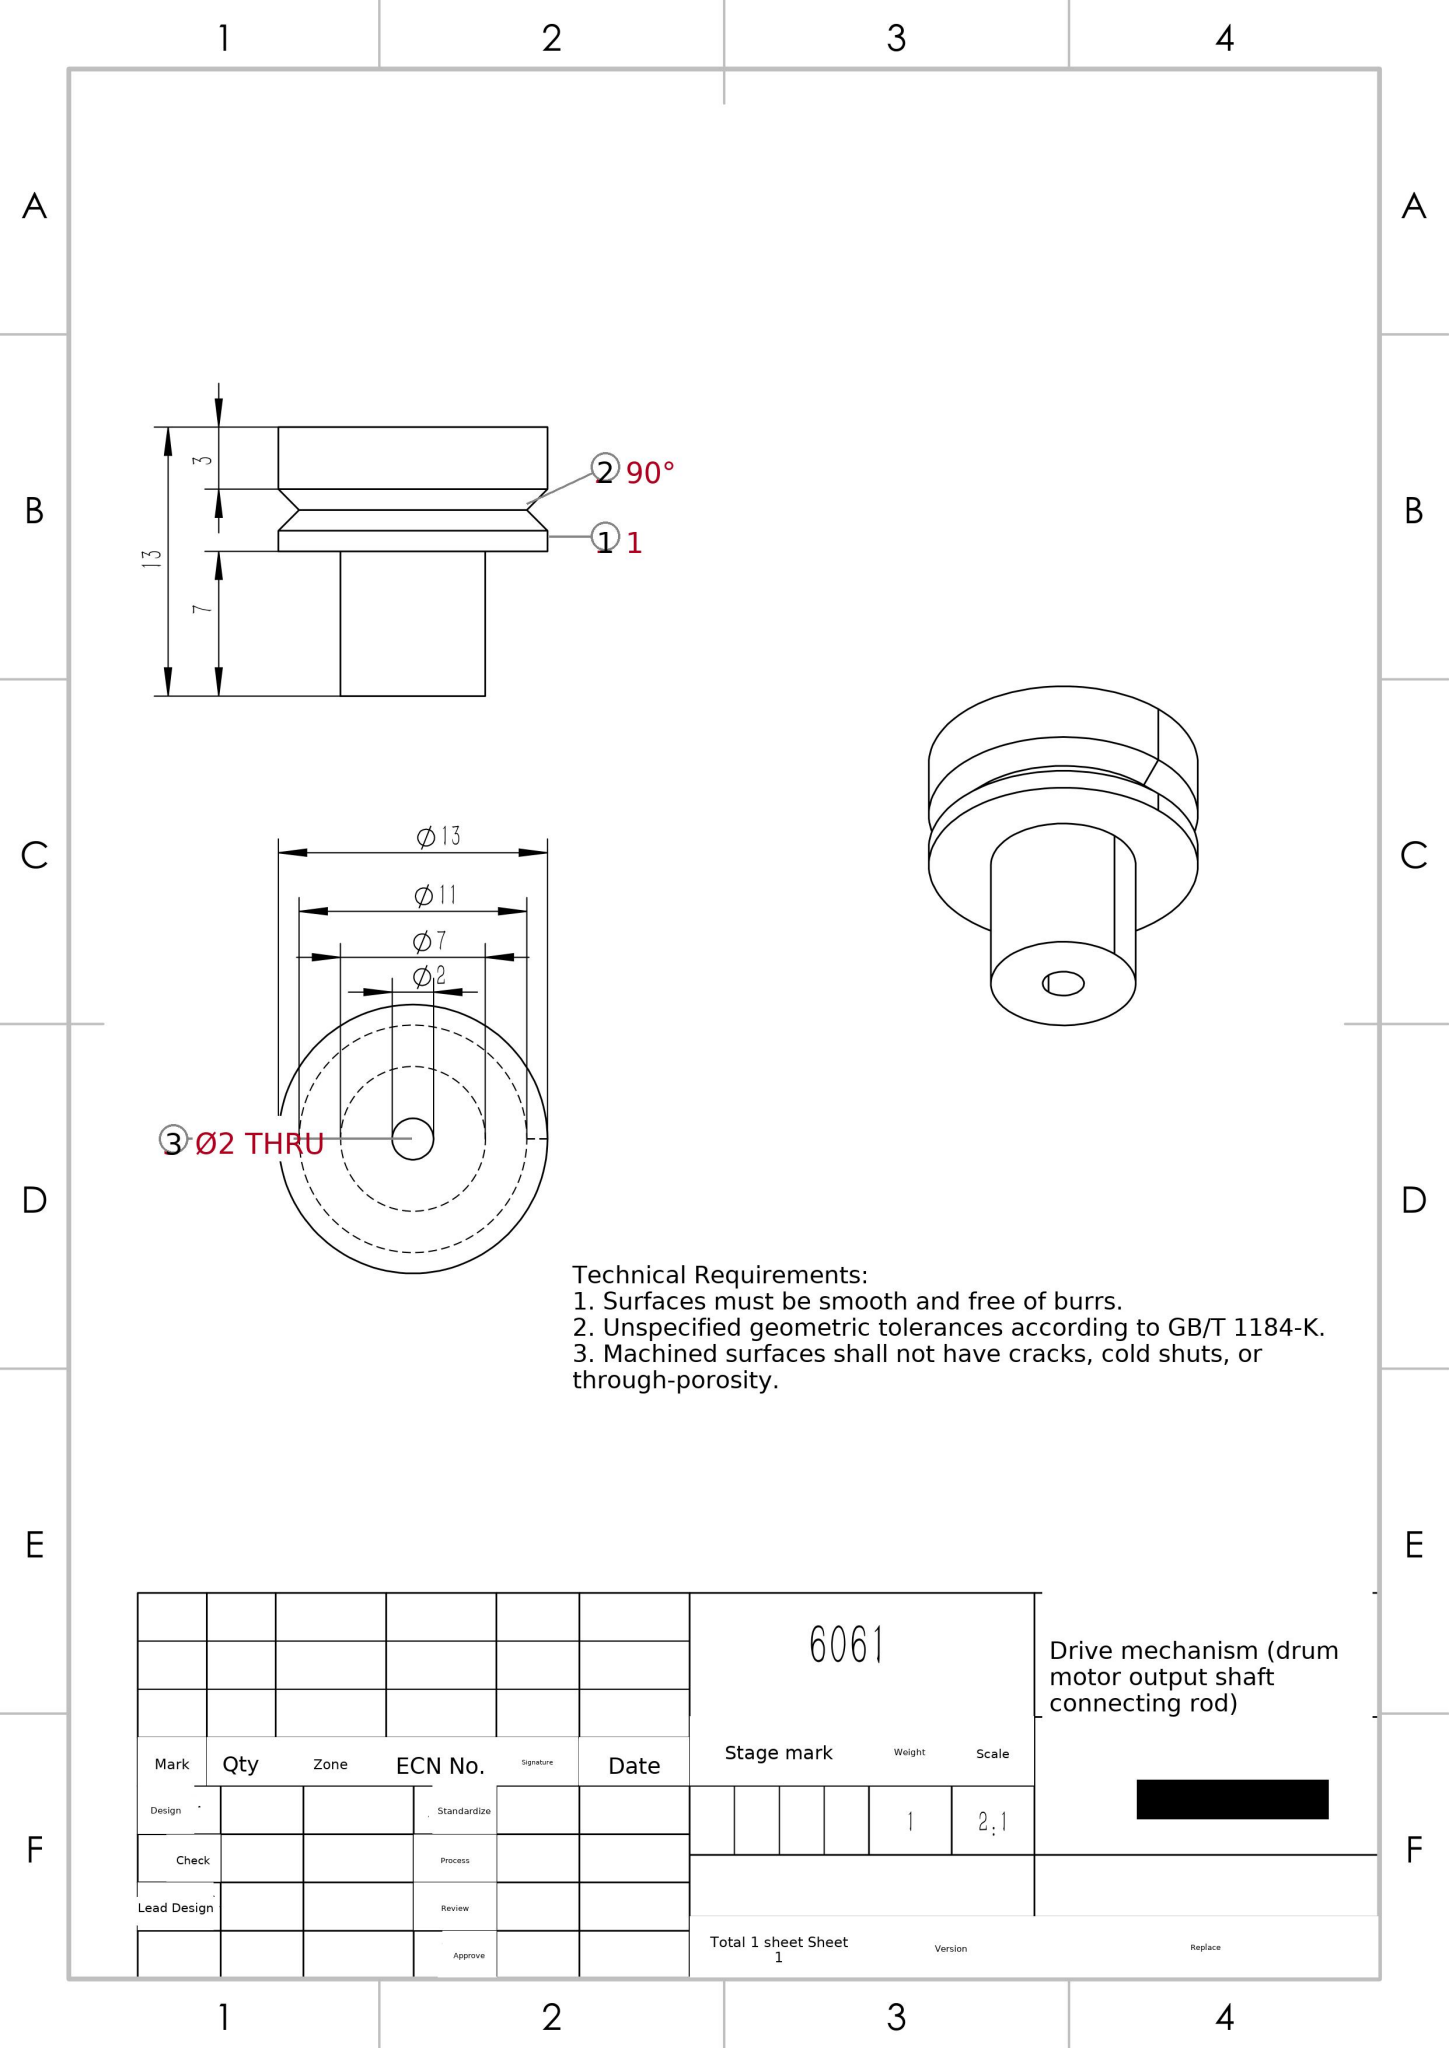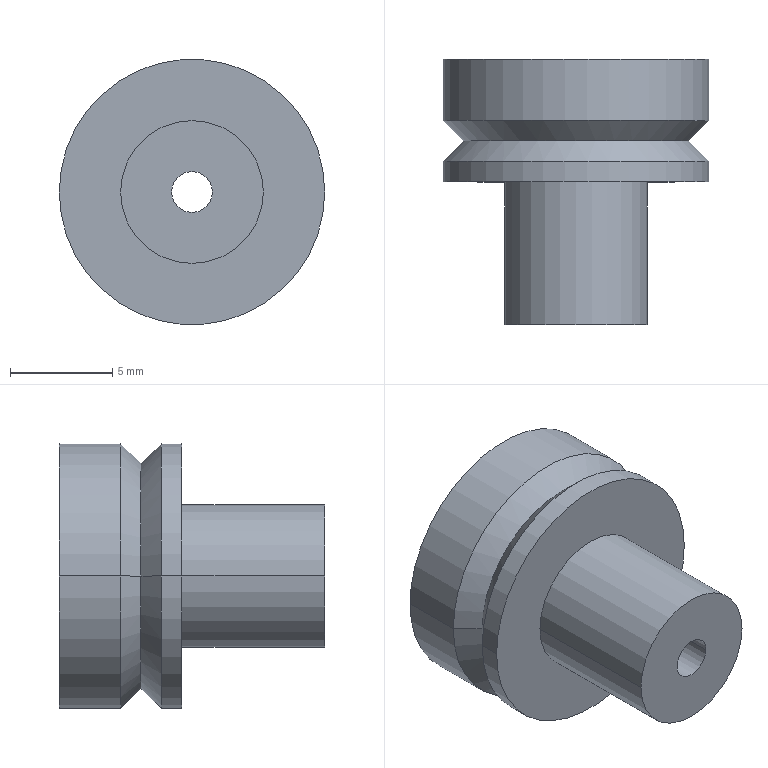Part | SolidWorks | mm | material 6061 | 1 solid | 15 faces | box 13 x 13 x 13 mm | volume 986 mm3 | cylinder 8 | cone 4 | plane 3 | commonest cylinder face diameters 13 x4 2 x2 7 x2
STEP:
#1=CARTESIAN_POINT('',(1.,-0.,0.));
#2=VERTEX_POINT('',#1);
#3=CARTESIAN_POINT('',(1.,13.,0.));
#4=VERTEX_POINT('',#3);
#5=CARTESIAN_POINT('',(1.,-0.,0.));
#6=DIRECTION('',(0.,1.,0.));
#7=VECTOR('',#6,1000.);
#8=LINE('',#5,#7);
#9=EDGE_CURVE('',#2,#4,#8,.T.);
#10=ORIENTED_EDGE('',*,*,#9,.F.);
#11=CARTESIAN_POINT('',(-1.,0.,0.));
#12=VERTEX_POINT('',#11);
#13=CARTESIAN_POINT('',(0.,0.,0.));
#14=DIRECTION('',(0.,1.,0.));
#15=DIRECTION('',(-1.,0.,0.));
#16=AXIS2_PLACEMENT_3D('',#13,#14,#15);
#17=CIRCLE('',#16,1.);
#18=EDGE_CURVE('',#12,#2,#17,.T.);
#19=ORIENTED_EDGE('',*,*,#18,.F.);
#20=CARTESIAN_POINT('',(-1.,13.,0.));
#21=VERTEX_POINT('',#20);
#22=CARTESIAN_POINT('',(-1.,0.,0.));
#23=DIRECTION('',(0.,1.,0.));
#24=VECTOR('',#23,1000.);
#25=LINE('',#22,#24);
#26=EDGE_CURVE('',#12,#21,#25,.T.);
#27=ORIENTED_EDGE('',*,*,#26,.T.);
#28=CARTESIAN_POINT('',(0.,13.,0.));
#29=DIRECTION('',(0.,1.,0.));
#30=DIRECTION('',(-1.,0.,0.));
#31=AXIS2_PLACEMENT_3D('',#28,#29,#30);
#32=CIRCLE('',#31,1.);
#33=EDGE_CURVE('',#21,#4,#32,.T.);
#34=ORIENTED_EDGE('',*,*,#33,.T.);
#35=EDGE_LOOP('',(#10,#19,#27,#34));
#36=FACE_OUTER_BOUND('',#35,.T.);
#37=CARTESIAN_POINT('',(0.,0.,0.));
#38=DIRECTION('',(0.,1.,0.));
#39=DIRECTION('',(-1.,0.,0.));
#40=AXIS2_PLACEMENT_3D('',#37,#38,#39);
#41=CYLINDRICAL_SURFACE('',#40,1.);
#42=ADVANCED_FACE('',(#36),#41,.F.);
#43=ORIENTED_EDGE('',*,*,#18,.T.);
#44=CARTESIAN_POINT('',(0.,0.,0.));
#45=DIRECTION('',(0.,1.,0.));
#46=DIRECTION('',(-1.,0.,0.));
#47=AXIS2_PLACEMENT_3D('',#44,#45,#46);
#48=CIRCLE('',#47,1.);
#49=EDGE_CURVE('',#2,#12,#48,.T.);
#50=ORIENTED_EDGE('',*,*,#49,.T.);
#51=EDGE_LOOP('',(#43,#50));
#52=FACE_BOUND('',#51,.T.);
#53=CARTESIAN_POINT('',(3.5,0.,0.));
#54=VERTEX_POINT('',#53);
#55=CARTESIAN_POINT('',(-3.5,0.,0.));
#56=VERTEX_POINT('',#55);
#57=CARTESIAN_POINT('',(0.,0.,0.));
#58=DIRECTION('',(-0.,-1.,0.));
#59=DIRECTION('',(1.,-0.,0.));
#60=AXIS2_PLACEMENT_3D('',#57,#58,#59);
#61=CIRCLE('',#60,3.5);
#62=EDGE_CURVE('',#54,#56,#61,.T.);
#63=ORIENTED_EDGE('',*,*,#62,.T.);
#64=CARTESIAN_POINT('',(0.,0.,0.));
#65=DIRECTION('',(-0.,-1.,0.));
#66=DIRECTION('',(1.,-0.,0.));
#67=AXIS2_PLACEMENT_3D('',#64,#65,#66);
#68=CIRCLE('',#67,3.5);
#69=EDGE_CURVE('',#56,#54,#68,.T.);
#70=ORIENTED_EDGE('',*,*,#69,.T.);
#71=EDGE_LOOP('',(#63,#70));
#72=FACE_OUTER_BOUND('',#71,.T.);
#73=CARTESIAN_POINT('',(3.5,-0.,0.));
#74=DIRECTION('',(-0.,-1.,0.));
#75=DIRECTION('',(-1.,0.,0.));
#76=AXIS2_PLACEMENT_3D('',#73,#74,#75);
#77=PLANE('',#76);
#78=ADVANCED_FACE('',(#52,#72),#77,.T.);
#79=CARTESIAN_POINT('',(-3.5,7.,0.));
#80=VERTEX_POINT('',#79);
#81=CARTESIAN_POINT('',(-3.5,0.,0.));
#82=DIRECTION('',(-0.,-1.,0.));
#83=VECTOR('',#82,1000.);
#84=LINE('',#81,#83);
#85=EDGE_CURVE('',#80,#56,#84,.T.);
#86=ORIENTED_EDGE('',*,*,#85,.F.);
#87=CARTESIAN_POINT('',(3.5,7.,0.));
#88=VERTEX_POINT('',#87);
#89=CARTESIAN_POINT('',(0.,7.,0.));
#90=DIRECTION('',(-0.,-1.,0.));
#91=DIRECTION('',(1.,-0.,0.));
#92=AXIS2_PLACEMENT_3D('',#89,#90,#91);
#93=CIRCLE('',#92,3.5);
#94=EDGE_CURVE('',#80,#88,#93,.T.);
#95=ORIENTED_EDGE('',*,*,#94,.T.);
#96=CARTESIAN_POINT('',(3.5,-0.,0.));
#97=DIRECTION('',(-0.,-1.,0.));
#98=VECTOR('',#97,1000.);
#99=LINE('',#96,#98);
#100=EDGE_CURVE('',#88,#54,#99,.T.);
#101=ORIENTED_EDGE('',*,*,#100,.T.);
#102=ORIENTED_EDGE('',*,*,#69,.F.);
#103=EDGE_LOOP('',(#86,#95,#101,#102));
#104=FACE_OUTER_BOUND('',#103,.T.);
#105=CARTESIAN_POINT('',(0.,0.,0.));
#106=DIRECTION('',(-0.,-1.,0.));
#107=DIRECTION('',(1.,-0.,0.));
#108=AXIS2_PLACEMENT_3D('',#105,#106,#107);
#109=CYLINDRICAL_SURFACE('',#108,3.5);
#110=ADVANCED_FACE('',(#104),#109,.T.);
#111=CARTESIAN_POINT('',(0.,7.,0.));
#112=DIRECTION('',(-0.,-1.,0.));
#113=DIRECTION('',(1.,-0.,0.));
#114=AXIS2_PLACEMENT_3D('',#111,#112,#113);
#115=CIRCLE('',#114,3.5);
#116=EDGE_CURVE('',#88,#80,#115,.T.);
#117=ORIENTED_EDGE('',*,*,#116,.F.);
#118=ORIENTED_EDGE('',*,*,#94,.F.);
#119=EDGE_LOOP('',(#117,#118));
#120=FACE_BOUND('',#119,.T.);
#121=CARTESIAN_POINT('',(6.5,7.,0.));
#122=VERTEX_POINT('',#121);
#123=CARTESIAN_POINT('',(-6.5,7.,0.));
#124=VERTEX_POINT('',#123);
#125=CARTESIAN_POINT('',(0.,7.,0.));
#126=DIRECTION('',(-0.,-1.,0.));
#127=DIRECTION('',(1.,-0.,0.));
#128=AXIS2_PLACEMENT_3D('',#125,#126,#127);
#129=CIRCLE('',#128,6.5);
#130=EDGE_CURVE('',#122,#124,#129,.T.);
#131=ORIENTED_EDGE('',*,*,#130,.T.);
#132=CARTESIAN_POINT('',(0.,7.,0.));
#133=DIRECTION('',(-0.,-1.,0.));
#134=DIRECTION('',(1.,-0.,0.));
#135=AXIS2_PLACEMENT_3D('',#132,#133,#134);
#136=CIRCLE('',#135,6.5);
#137=EDGE_CURVE('',#124,#122,#136,.T.);
#138=ORIENTED_EDGE('',*,*,#137,.T.);
#139=EDGE_LOOP('',(#131,#138));
#140=FACE_OUTER_BOUND('',#139,.T.);
#141=CARTESIAN_POINT('',(6.5,7.,0.));
#142=DIRECTION('',(-0.,-1.,0.));
#143=DIRECTION('',(-1.,0.,0.));
#144=AXIS2_PLACEMENT_3D('',#141,#142,#143);
#145=PLANE('',#144);
#146=ADVANCED_FACE('',(#120,#140),#145,.T.);
#147=CARTESIAN_POINT('',(-6.5,8.,0.));
#148=VERTEX_POINT('',#147);
#149=CARTESIAN_POINT('',(-6.5,0.,0.));
#150=DIRECTION('',(-0.,-1.,0.));
#151=VECTOR('',#150,1000.);
#152=LINE('',#149,#151);
#153=EDGE_CURVE('',#148,#124,#152,.T.);
#154=ORIENTED_EDGE('',*,*,#153,.F.);
#155=CARTESIAN_POINT('',(6.5,8.,0.));
#156=VERTEX_POINT('',#155);
#157=CARTESIAN_POINT('',(0.,8.,0.));
#158=DIRECTION('',(-0.,-1.,0.));
#159=DIRECTION('',(1.,-0.,0.));
#160=AXIS2_PLACEMENT_3D('',#157,#158,#159);
#161=CIRCLE('',#160,6.5);
#162=EDGE_CURVE('',#148,#156,#161,.T.);
#163=ORIENTED_EDGE('',*,*,#162,.T.);
#164=CARTESIAN_POINT('',(6.5,-0.,0.));
#165=DIRECTION('',(-0.,-1.,0.));
#166=VECTOR('',#165,1000.);
#167=LINE('',#164,#166);
#168=EDGE_CURVE('',#156,#122,#167,.T.);
#169=ORIENTED_EDGE('',*,*,#168,.T.);
#170=ORIENTED_EDGE('',*,*,#137,.F.);
#171=EDGE_LOOP('',(#154,#163,#169,#170));
#172=FACE_OUTER_BOUND('',#171,.T.);
#173=CARTESIAN_POINT('',(0.,0.,0.));
#174=DIRECTION('',(-0.,-1.,0.));
#175=DIRECTION('',(1.,-0.,0.));
#176=AXIS2_PLACEMENT_3D('',#173,#174,#175);
#177=CYLINDRICAL_SURFACE('',#176,6.5);
#178=ADVANCED_FACE('',(#172),#177,.T.);
#179=CARTESIAN_POINT('',(-5.5,9.,0.));
#180=VERTEX_POINT('',#179);
#181=CARTESIAN_POINT('',(-6.5,8.,0.));
#182=DIRECTION('',(-0.7071,-0.7071,0.));
#183=VECTOR('',#182,1000.);
#184=LINE('',#181,#183);
#185=EDGE_CURVE('',#180,#148,#184,.T.);
#186=ORIENTED_EDGE('',*,*,#185,.F.);
#187=CARTESIAN_POINT('',(5.5,9.,0.));
#188=VERTEX_POINT('',#187);
#189=CARTESIAN_POINT('',(0.,9.,0.));
#190=DIRECTION('',(0.,-1.,0.));
#191=DIRECTION('',(1.,0.,0.));
#192=AXIS2_PLACEMENT_3D('',#189,#190,#191);
#193=CIRCLE('',#192,5.5);
#194=EDGE_CURVE('',#180,#188,#193,.T.);
#195=ORIENTED_EDGE('',*,*,#194,.T.);
#196=CARTESIAN_POINT('',(6.5,8.,0.));
#197=DIRECTION('',(0.7071,-0.7071,0.));
#198=VECTOR('',#197,1000.);
#199=LINE('',#196,#198);
#200=EDGE_CURVE('',#188,#156,#199,.T.);
#201=ORIENTED_EDGE('',*,*,#200,.T.);
#202=ORIENTED_EDGE('',*,*,#162,.F.);
#203=EDGE_LOOP('',(#186,#195,#201,#202));
#204=FACE_OUTER_BOUND('',#203,.T.);
#205=CARTESIAN_POINT('',(0.,8.,0.));
#206=DIRECTION('',(-0.,-1.,0.));
#207=DIRECTION('',(1.,-0.,0.));
#208=AXIS2_PLACEMENT_3D('',#205,#206,#207);
#209=CONICAL_SURFACE('',#208,6.5,0.7854);
#210=ADVANCED_FACE('',(#204),#209,.T.);
#211=CARTESIAN_POINT('',(6.5,10.,0.));
#212=VERTEX_POINT('',#211);
#213=CARTESIAN_POINT('',(5.5,9.,0.));
#214=DIRECTION('',(0.7071,0.7071,0.));
#215=VECTOR('',#214,1000.);
#216=LINE('',#213,#215);
#217=EDGE_CURVE('',#188,#212,#216,.T.);
#218=ORIENTED_EDGE('',*,*,#217,.F.);
#219=ORIENTED_EDGE('',*,*,#194,.F.);
#220=CARTESIAN_POINT('',(-6.5,10.,0.));
#221=VERTEX_POINT('',#220);
#222=CARTESIAN_POINT('',(-5.5,9.,0.));
#223=DIRECTION('',(-0.7071,0.7071,0.));
#224=VECTOR('',#223,1000.);
#225=LINE('',#222,#224);
#226=EDGE_CURVE('',#180,#221,#225,.T.);
#227=ORIENTED_EDGE('',*,*,#226,.T.);
#228=CARTESIAN_POINT('',(0.,10.,0.));
#229=DIRECTION('',(-0.,-1.,0.));
#230=DIRECTION('',(1.,-0.,0.));
#231=AXIS2_PLACEMENT_3D('',#228,#229,#230);
#232=CIRCLE('',#231,6.5);
#233=EDGE_CURVE('',#221,#212,#232,.T.);
#234=ORIENTED_EDGE('',*,*,#233,.T.);
#235=EDGE_LOOP('',(#218,#219,#227,#234));
#236=FACE_OUTER_BOUND('',#235,.T.);
#237=CARTESIAN_POINT('',(0.,9.,0.));
#238=DIRECTION('',(0.,1.,0.));
#239=DIRECTION('',(-1.,0.,0.));
#240=AXIS2_PLACEMENT_3D('',#237,#238,#239);
#241=CONICAL_SURFACE('',#240,5.5,0.7854);
#242=ADVANCED_FACE('',(#236),#241,.T.);
#243=CARTESIAN_POINT('',(-6.5,13.,0.));
#244=VERTEX_POINT('',#243);
#245=CARTESIAN_POINT('',(-6.5,0.,0.));
#246=DIRECTION('',(-0.,-1.,0.));
#247=VECTOR('',#246,1000.);
#248=LINE('',#245,#247);
#249=EDGE_CURVE('',#244,#221,#248,.T.);
#250=ORIENTED_EDGE('',*,*,#249,.F.);
#251=CARTESIAN_POINT('',(6.5,13.,0.));
#252=VERTEX_POINT('',#251);
#253=CARTESIAN_POINT('',(0.,13.,0.));
#254=DIRECTION('',(-0.,-1.,0.));
#255=DIRECTION('',(1.,-0.,0.));
#256=AXIS2_PLACEMENT_3D('',#253,#254,#255);
#257=CIRCLE('',#256,6.5);
#258=EDGE_CURVE('',#244,#252,#257,.T.);
#259=ORIENTED_EDGE('',*,*,#258,.T.);
#260=CARTESIAN_POINT('',(6.5,-0.,0.));
#261=DIRECTION('',(-0.,-1.,0.));
#262=VECTOR('',#261,1000.);
#263=LINE('',#260,#262);
#264=EDGE_CURVE('',#252,#212,#263,.T.);
#265=ORIENTED_EDGE('',*,*,#264,.T.);
#266=ORIENTED_EDGE('',*,*,#233,.F.);
#267=EDGE_LOOP('',(#250,#259,#265,#266));
#268=FACE_OUTER_BOUND('',#267,.T.);
#269=CARTESIAN_POINT('',(0.,0.,0.));
#270=DIRECTION('',(-0.,-1.,0.));
#271=DIRECTION('',(1.,-0.,0.));
#272=AXIS2_PLACEMENT_3D('',#269,#270,#271);
#273=CYLINDRICAL_SURFACE('',#272,6.5);
#274=ADVANCED_FACE('',(#268),#273,.T.);
#275=ORIENTED_EDGE('',*,*,#33,.F.);
#276=CARTESIAN_POINT('',(0.,13.,0.));
#277=DIRECTION('',(0.,1.,0.));
#278=DIRECTION('',(-1.,0.,0.));
#279=AXIS2_PLACEMENT_3D('',#276,#277,#278);
#280=CIRCLE('',#279,1.);
#281=EDGE_CURVE('',#4,#21,#280,.T.);
#282=ORIENTED_EDGE('',*,*,#281,.F.);
#283=EDGE_LOOP('',(#275,#282));
#284=FACE_BOUND('',#283,.T.);
#285=CARTESIAN_POINT('',(0.,13.,0.));
#286=DIRECTION('',(-0.,-1.,0.));
#287=DIRECTION('',(1.,-0.,0.));
#288=AXIS2_PLACEMENT_3D('',#285,#286,#287);
#289=CIRCLE('',#288,6.5);
#290=EDGE_CURVE('',#252,#244,#289,.T.);
#291=ORIENTED_EDGE('',*,*,#290,.F.);
#292=ORIENTED_EDGE('',*,*,#258,.F.);
#293=EDGE_LOOP('',(#291,#292));
#294=FACE_OUTER_BOUND('',#293,.T.);
#295=CARTESIAN_POINT('',(0.,13.,0.));
#296=DIRECTION('',(0.,1.,0.));
#297=DIRECTION('',(1.,-0.,0.));
#298=AXIS2_PLACEMENT_3D('',#295,#296,#297);
#299=PLANE('',#298);
#300=ADVANCED_FACE('',(#284,#294),#299,.T.);
#301=ORIENTED_EDGE('',*,*,#290,.T.);
#302=ORIENTED_EDGE('',*,*,#249,.T.);
#303=CARTESIAN_POINT('',(0.,10.,0.));
#304=DIRECTION('',(-0.,-1.,0.));
#305=DIRECTION('',(1.,-0.,0.));
#306=AXIS2_PLACEMENT_3D('',#303,#304,#305);
#307=CIRCLE('',#306,6.5);
#308=EDGE_CURVE('',#212,#221,#307,.T.);
#309=ORIENTED_EDGE('',*,*,#308,.F.);
#310=ORIENTED_EDGE('',*,*,#264,.F.);
#311=EDGE_LOOP('',(#301,#302,#309,#310));
#312=FACE_OUTER_BOUND('',#311,.T.);
#313=CARTESIAN_POINT('',(0.,0.,0.));
#314=DIRECTION('',(-0.,-1.,0.));
#315=DIRECTION('',(1.,-0.,0.));
#316=AXIS2_PLACEMENT_3D('',#313,#314,#315);
#317=CYLINDRICAL_SURFACE('',#316,6.5);
#318=ADVANCED_FACE('',(#312),#317,.T.);
#319=CARTESIAN_POINT('',(0.,9.,0.));
#320=DIRECTION('',(0.,-1.,0.));
#321=DIRECTION('',(1.,0.,0.));
#322=AXIS2_PLACEMENT_3D('',#319,#320,#321);
#323=CIRCLE('',#322,5.5);
#324=EDGE_CURVE('',#188,#180,#323,.T.);
#325=ORIENTED_EDGE('',*,*,#324,.F.);
#326=ORIENTED_EDGE('',*,*,#217,.T.);
#327=ORIENTED_EDGE('',*,*,#308,.T.);
#328=ORIENTED_EDGE('',*,*,#226,.F.);
#329=EDGE_LOOP('',(#325,#326,#327,#328));
#330=FACE_OUTER_BOUND('',#329,.T.);
#331=CARTESIAN_POINT('',(0.,9.,0.));
#332=DIRECTION('',(0.,1.,0.));
#333=DIRECTION('',(-1.,0.,0.));
#334=AXIS2_PLACEMENT_3D('',#331,#332,#333);
#335=CONICAL_SURFACE('',#334,5.5,0.7854);
#336=ADVANCED_FACE('',(#330),#335,.T.);
#337=ORIENTED_EDGE('',*,*,#324,.T.);
#338=ORIENTED_EDGE('',*,*,#185,.T.);
#339=CARTESIAN_POINT('',(0.,8.,0.));
#340=DIRECTION('',(-0.,-1.,0.));
#341=DIRECTION('',(1.,-0.,0.));
#342=AXIS2_PLACEMENT_3D('',#339,#340,#341);
#343=CIRCLE('',#342,6.5);
#344=EDGE_CURVE('',#156,#148,#343,.T.);
#345=ORIENTED_EDGE('',*,*,#344,.F.);
#346=ORIENTED_EDGE('',*,*,#200,.F.);
#347=EDGE_LOOP('',(#337,#338,#345,#346));
#348=FACE_OUTER_BOUND('',#347,.T.);
#349=CARTESIAN_POINT('',(0.,8.,0.));
#350=DIRECTION('',(-0.,-1.,0.));
#351=DIRECTION('',(1.,-0.,0.));
#352=AXIS2_PLACEMENT_3D('',#349,#350,#351);
#353=CONICAL_SURFACE('',#352,6.5,0.7854);
#354=ADVANCED_FACE('',(#348),#353,.T.);
#355=ORIENTED_EDGE('',*,*,#344,.T.);
#356=ORIENTED_EDGE('',*,*,#153,.T.);
#357=ORIENTED_EDGE('',*,*,#130,.F.);
#358=ORIENTED_EDGE('',*,*,#168,.F.);
#359=EDGE_LOOP('',(#355,#356,#357,#358));
#360=FACE_OUTER_BOUND('',#359,.T.);
#361=CARTESIAN_POINT('',(0.,0.,0.));
#362=DIRECTION('',(-0.,-1.,0.));
#363=DIRECTION('',(1.,-0.,0.));
#364=AXIS2_PLACEMENT_3D('',#361,#362,#363);
#365=CYLINDRICAL_SURFACE('',#364,6.5);
#366=ADVANCED_FACE('',(#360),#365,.T.);
#367=ORIENTED_EDGE('',*,*,#116,.T.);
#368=ORIENTED_EDGE('',*,*,#85,.T.);
#369=ORIENTED_EDGE('',*,*,#62,.F.);
#370=ORIENTED_EDGE('',*,*,#100,.F.);
#371=EDGE_LOOP('',(#367,#368,#369,#370));
#372=FACE_OUTER_BOUND('',#371,.T.);
#373=CARTESIAN_POINT('',(0.,0.,0.));
#374=DIRECTION('',(-0.,-1.,0.));
#375=DIRECTION('',(1.,-0.,0.));
#376=AXIS2_PLACEMENT_3D('',#373,#374,#375);
#377=CYLINDRICAL_SURFACE('',#376,3.5);
#378=ADVANCED_FACE('',(#372),#377,.T.);
#379=ORIENTED_EDGE('',*,*,#49,.F.);
#380=ORIENTED_EDGE('',*,*,#9,.T.);
#381=ORIENTED_EDGE('',*,*,#281,.T.);
#382=ORIENTED_EDGE('',*,*,#26,.F.);
#383=EDGE_LOOP('',(#379,#380,#381,#382));
#384=FACE_OUTER_BOUND('',#383,.T.);
#385=CARTESIAN_POINT('',(0.,0.,0.));
#386=DIRECTION('',(0.,1.,0.));
#387=DIRECTION('',(-1.,0.,0.));
#388=AXIS2_PLACEMENT_3D('',#385,#386,#387);
#389=CYLINDRICAL_SURFACE('',#388,1.);
#390=ADVANCED_FACE('',(#384),#389,.F.);
#391=CLOSED_SHELL('',(#42,#78,#110,#146,#178,#210,#242,#274,#300,#318,#336,#354,#366,#378,#390));
#392=MANIFOLD_SOLID_BREP('',#391);
#393=CARTESIAN_POINT('',(0.,0.,0.));
#394=DIRECTION('',(0.,0.,1.));
#395=DIRECTION('',(1.,0.,0.));
#396=AXIS2_PLACEMENT_3D('',#393,#394,#395);
#397=(LENGTH_UNIT()NAMED_UNIT(*)SI_UNIT(.MILLI.,.METRE.));
#398=UNCERTAINTY_MEASURE_WITH_UNIT(LENGTH_MEASURE(0.00001),#397,'','');
#399=(NAMED_UNIT(*)PLANE_ANGLE_UNIT()SI_UNIT($,.RADIAN.));
#400=(NAMED_UNIT(*)SI_UNIT($,.STERADIAN.)SOLID_ANGLE_UNIT());
#401=(GEOMETRIC_REPRESENTATION_CONTEXT(3)GLOBAL_UNCERTAINTY_ASSIGNED_CONTEXT((#398))GLOBAL_UNIT_ASSIGNED_CONTEXT((#397,#399,#400))REPRESENTATION_CONTEXT('',''));
#402=ADVANCED_BREP_SHAPE_REPRESENTATION('',(#392,#396),#401);